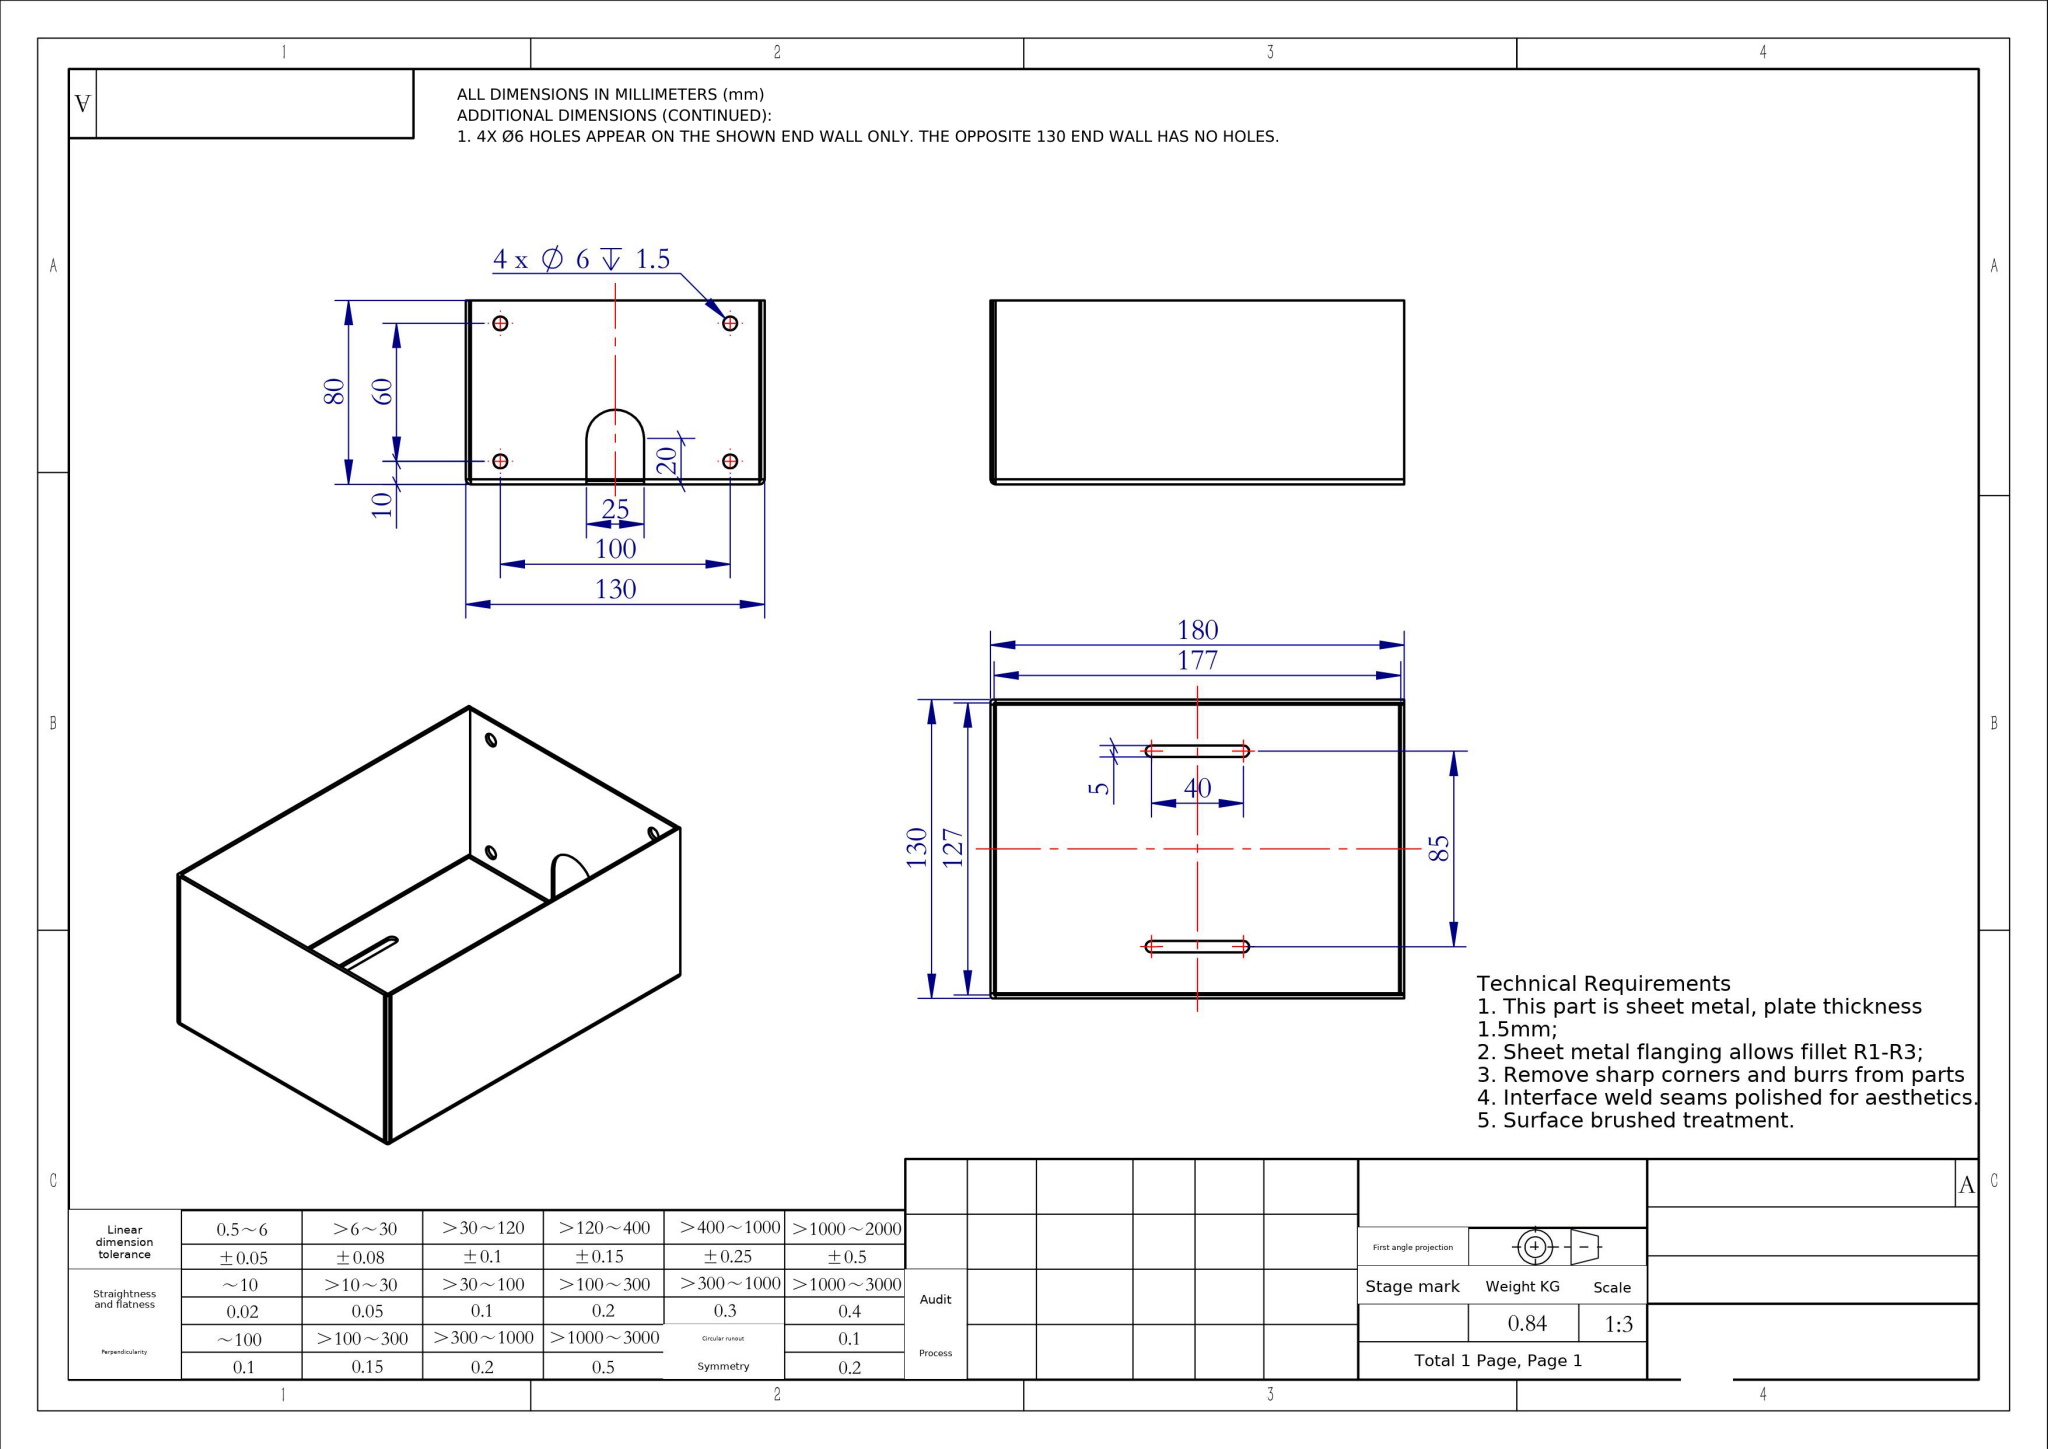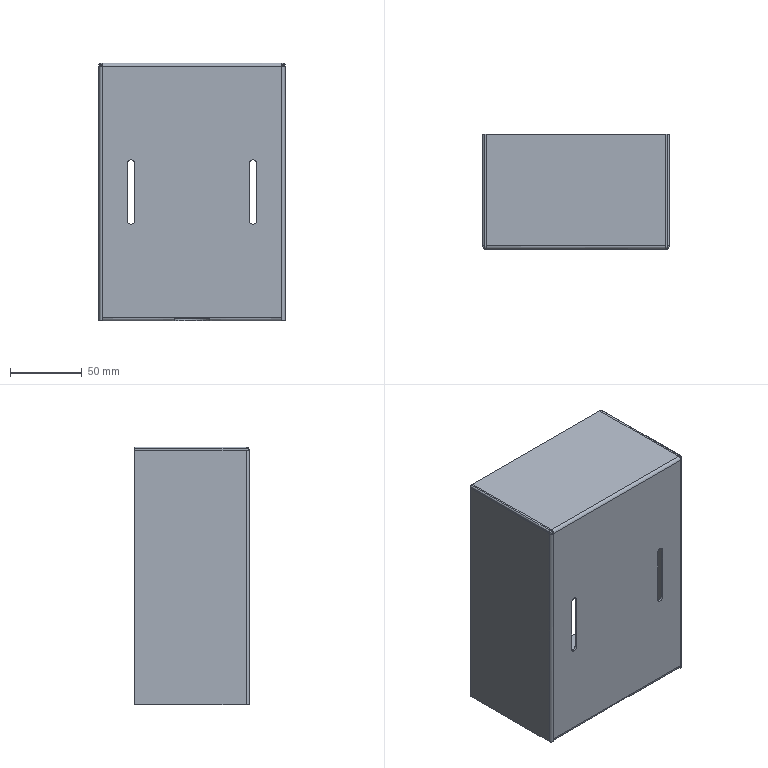Part | NX | mm | 1 solid | 76 faces | box 130 x 80 x 180 mm | volume 104672 mm3 | plane 41 | cylinder 24 | spline 11 | commonest cylinder face diameters 6 x8 5 x6 4.473 x4 1.473 x4 2 x2